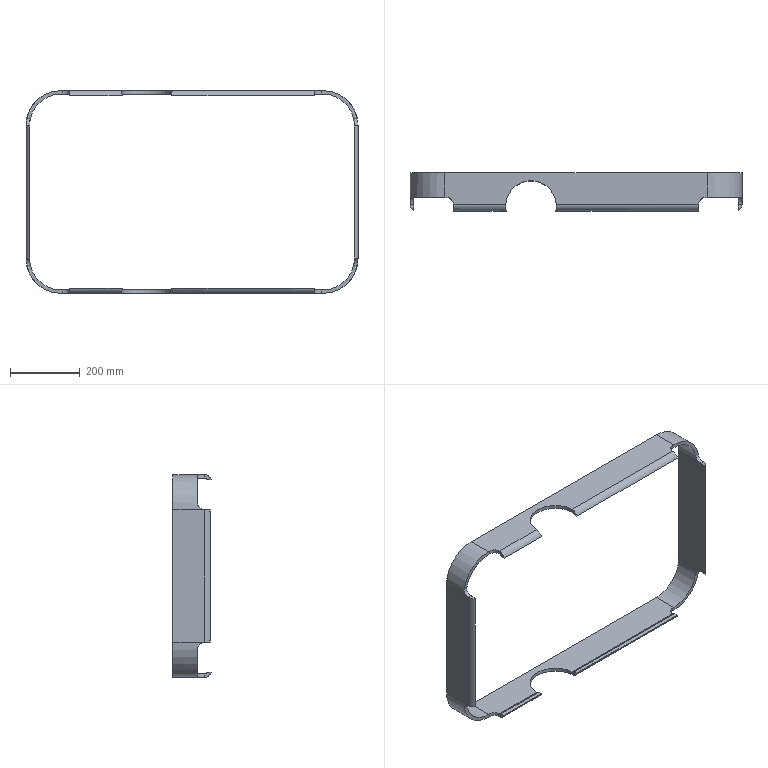Component | SolidWorks | Part27-1 | 1 solid | 65 faces | volume 2587821 mm3 | cylinder 40 | plane 25 | commonest cylinder face diameters 40 x14 180 x8 20 x8 145 x6 200 x4